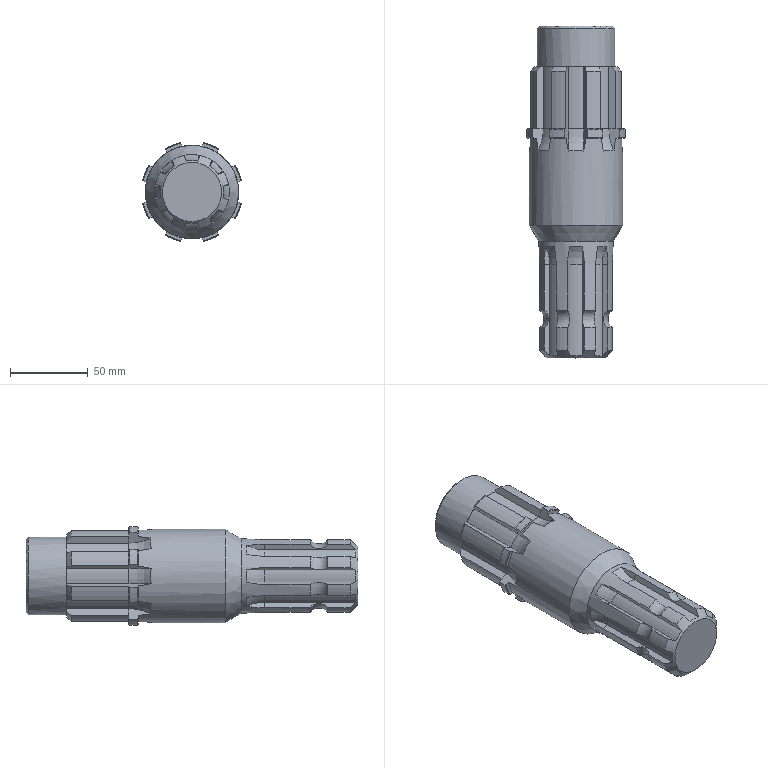Component | NX | UPPER_SHAFT | 1 solid | 177 faces | volume 455808 mm3 | cone 59 | plane 51 | cylinder 43 | torus 24 | commonest cylinder face diameters 48 x9 60 x9 65 x8 50.5 x8 40.5 x8 50 x1